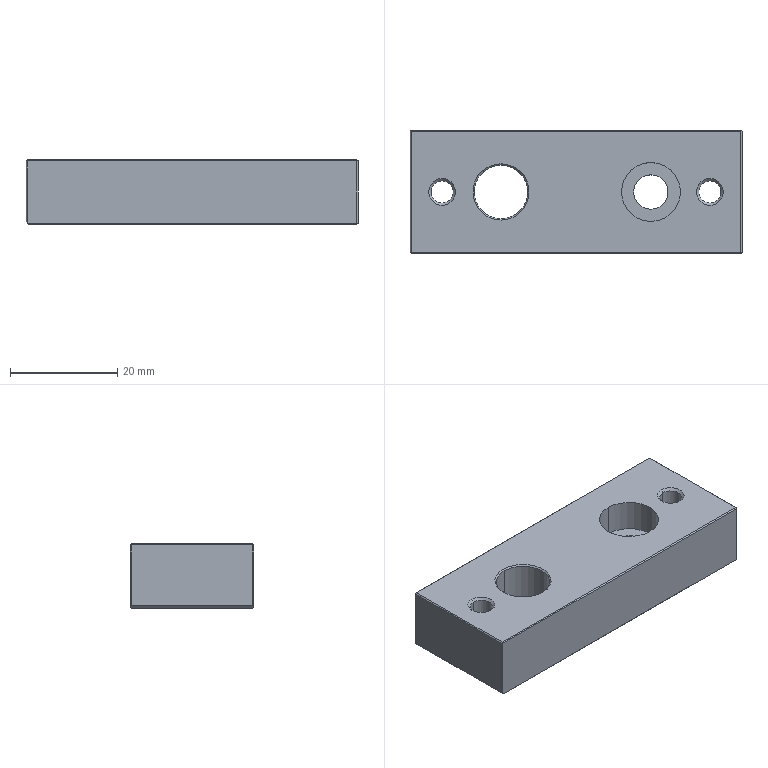Component | SolidWorks | TR-20x75-S-GN-1 (0)-3_TR-20x75-SBaffle-1 | 1 solid | 65 faces | volume 14812 mm3 | plane 27 | cone 22 | cylinder 16 | commonest cylinder face diameters 4.134 x4 3.242 x4 6.4 x2 10 x2 8 x2 11 x2